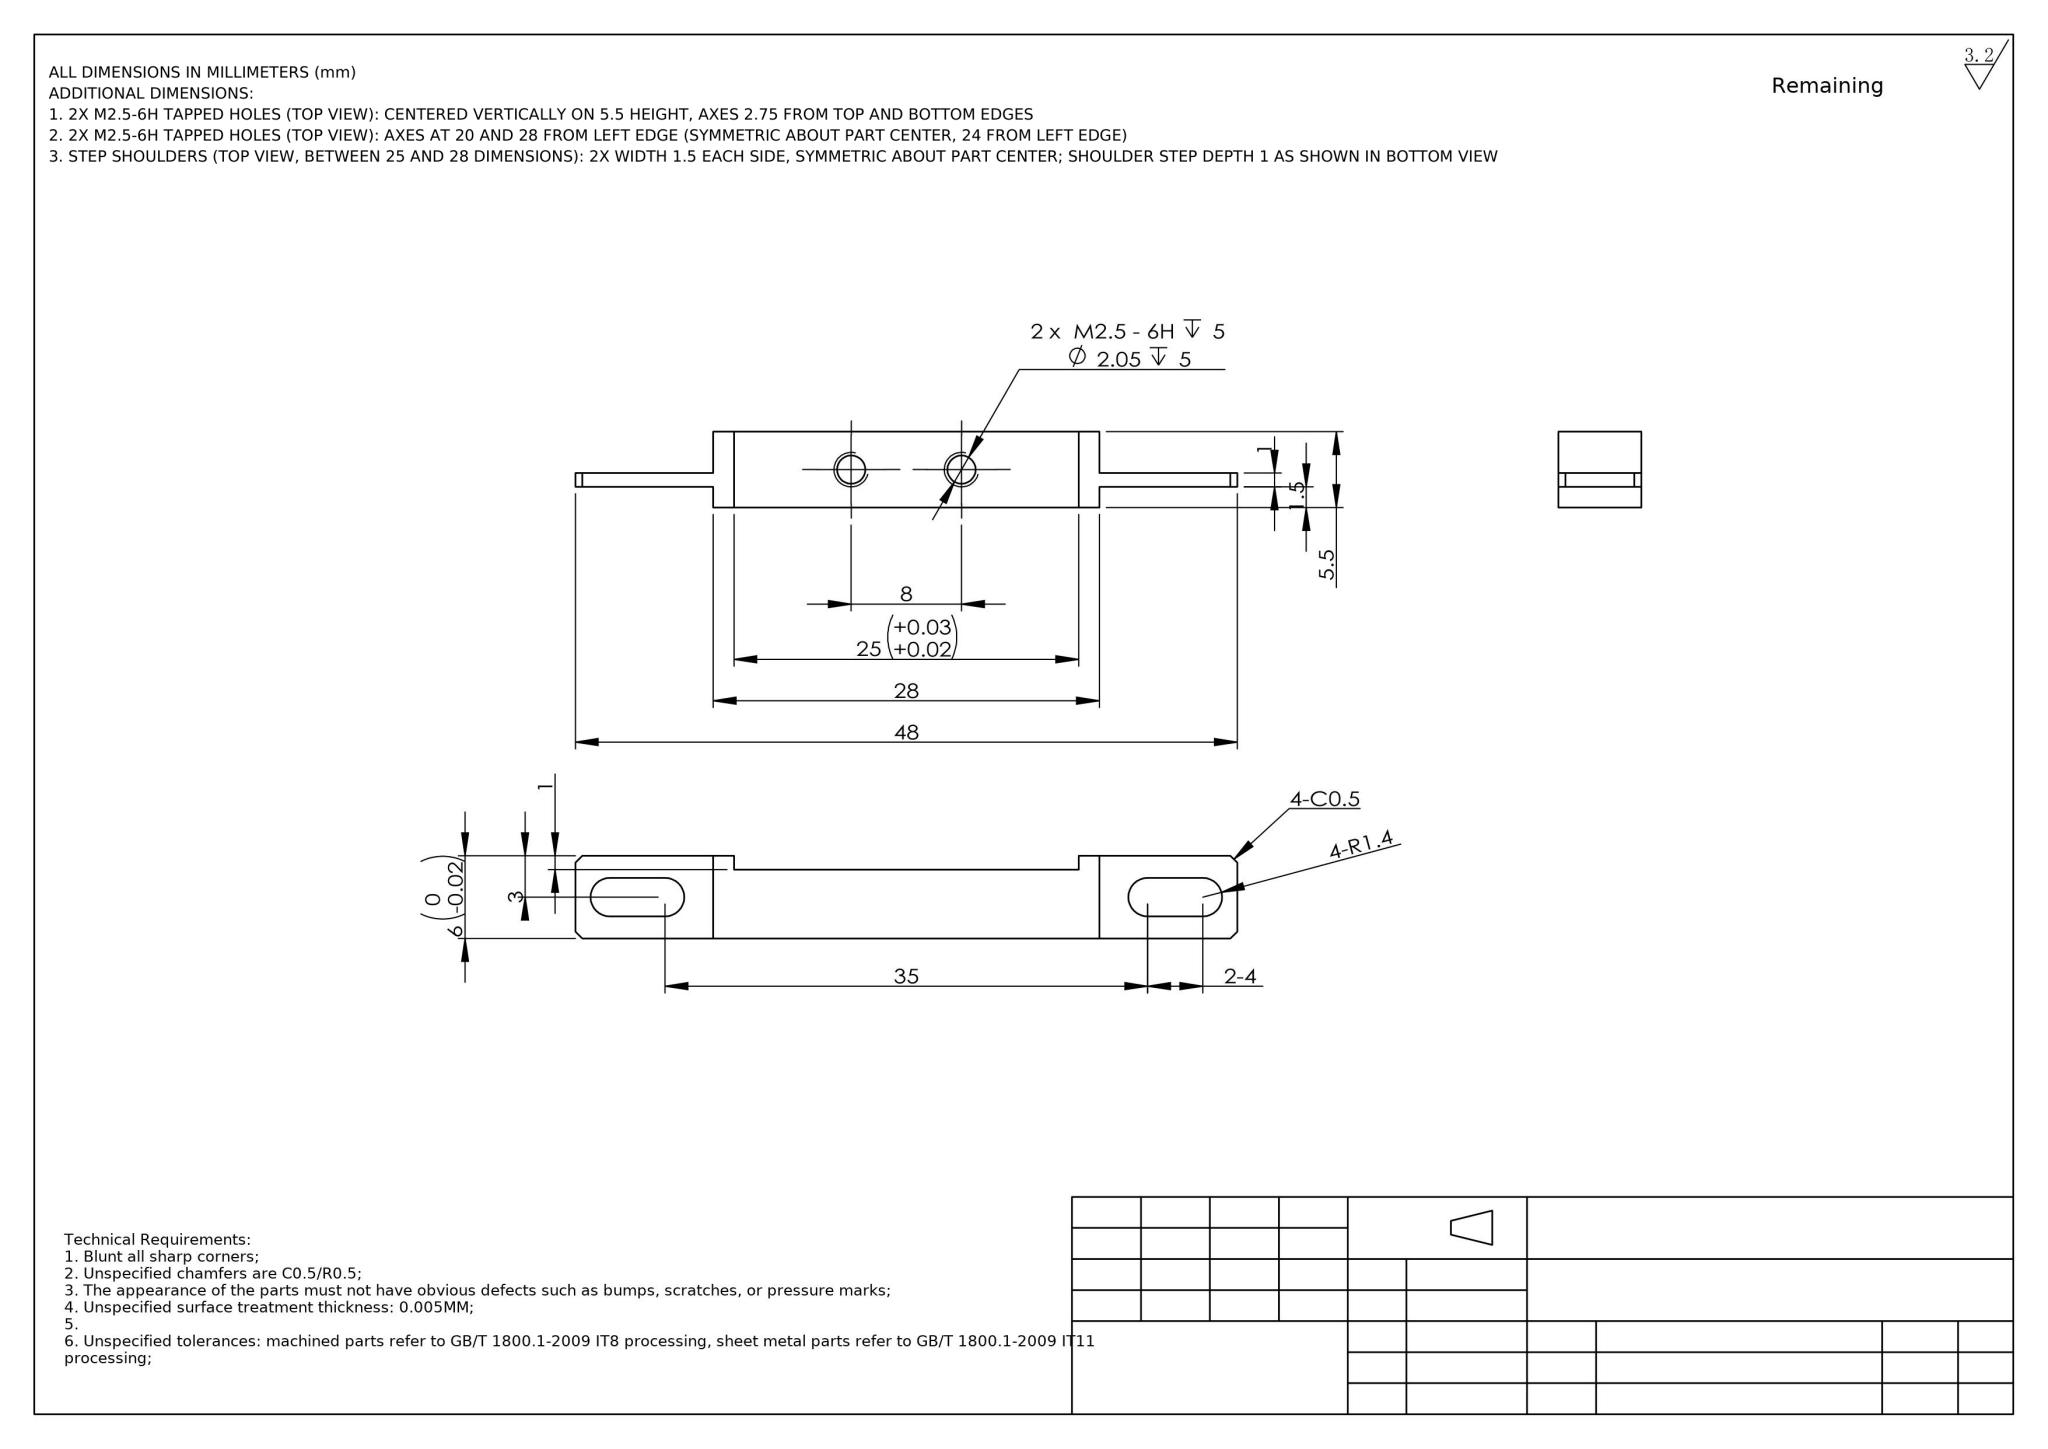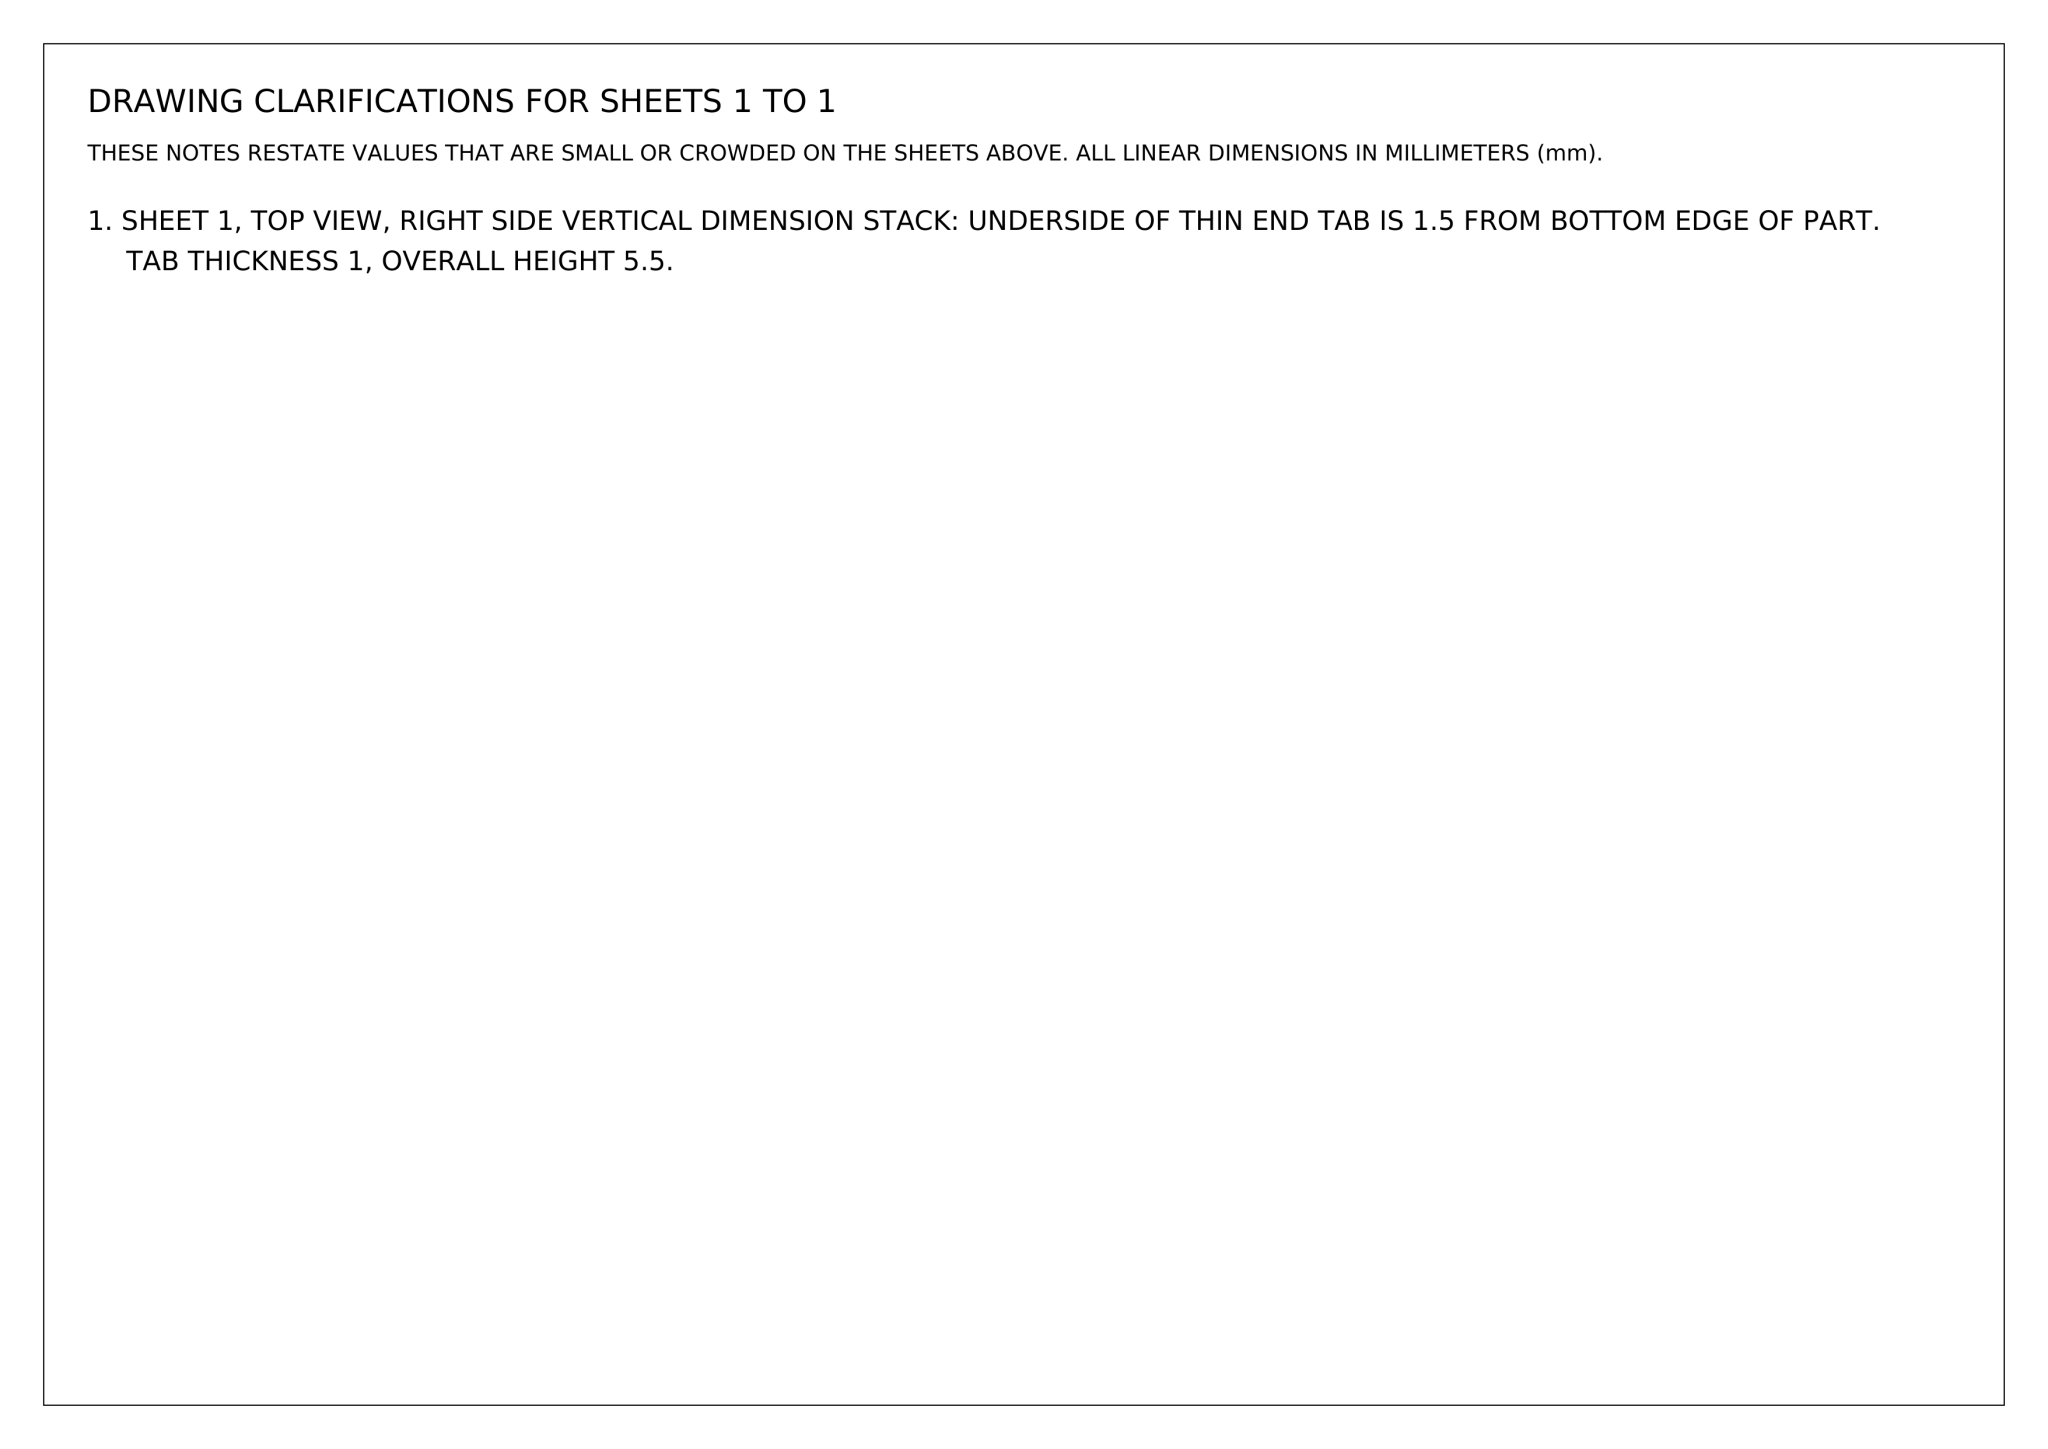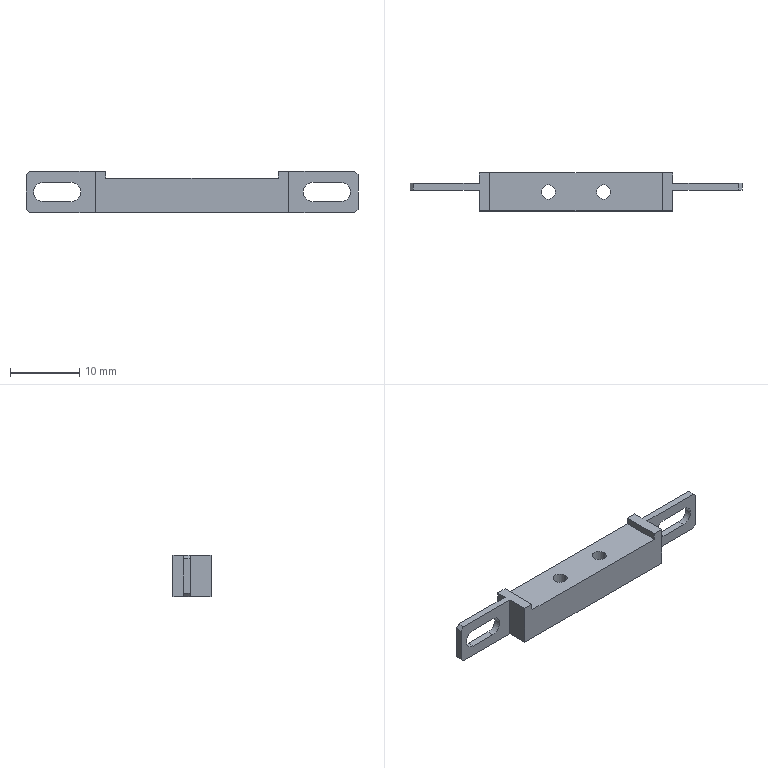Part | NX | mm | 1 solid | 34 faces | box 48 x 5.5 x 6 mm | volume 838 mm3 | plane 26 | cylinder 8 | commonest cylinder face diameters 2.05 x4 2.8 x4